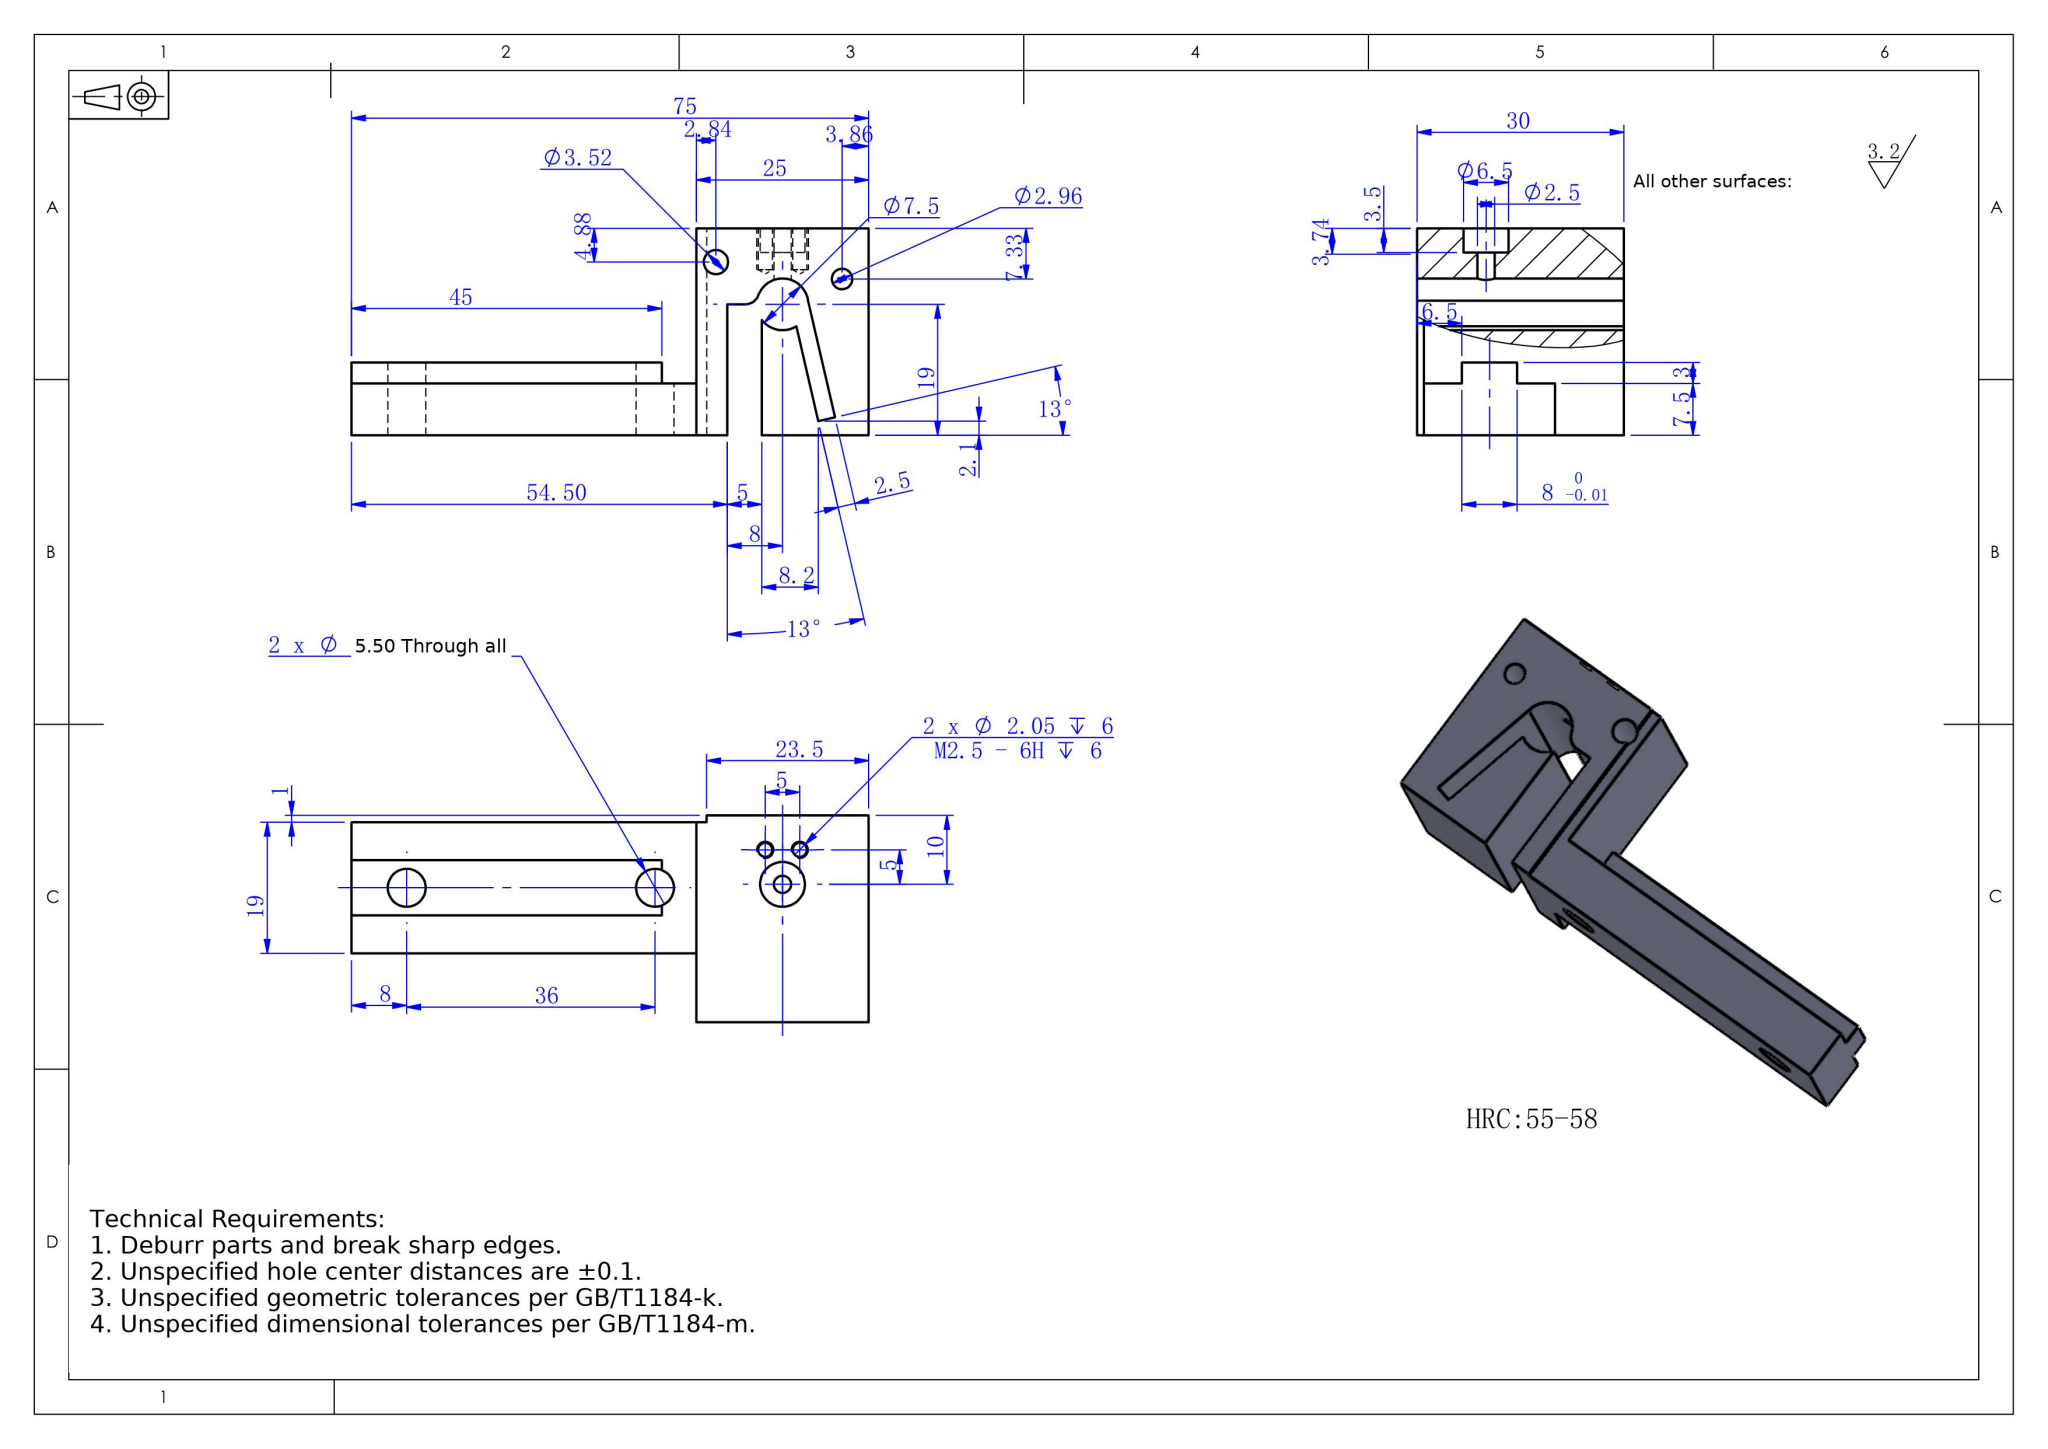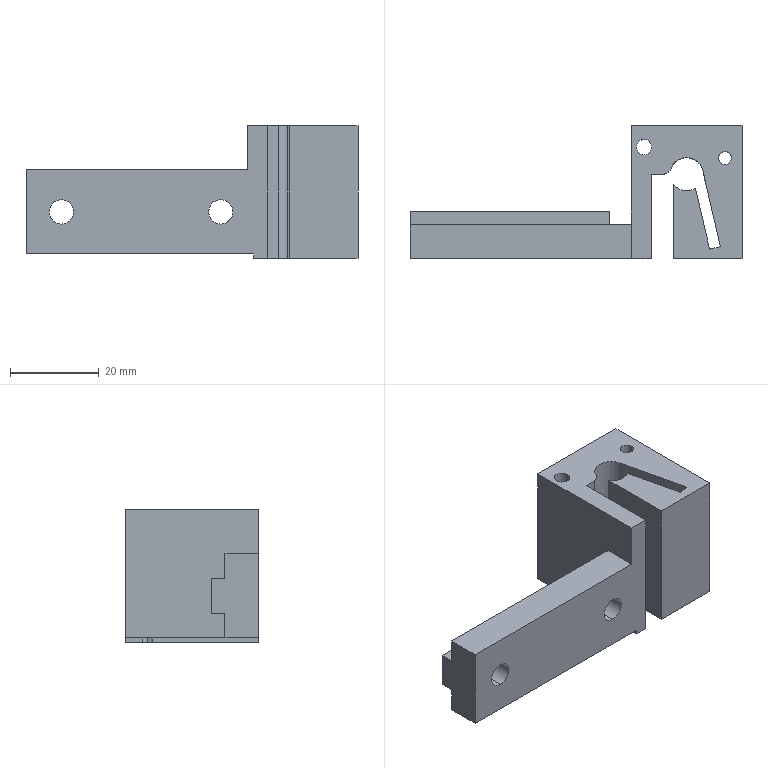Part | SolidWorks | mm | 1 solid | 48 faces | box 75 x 30 x 30 mm | volume 24266 mm3 | plane 25 | cylinder 19 | cone 4 | commonest cylinder face diameters 2.05 x4 5.5 x4 2.964 x2 3.521 x2 6.5 x2 2.5 x2 7.5 x2 4 x1